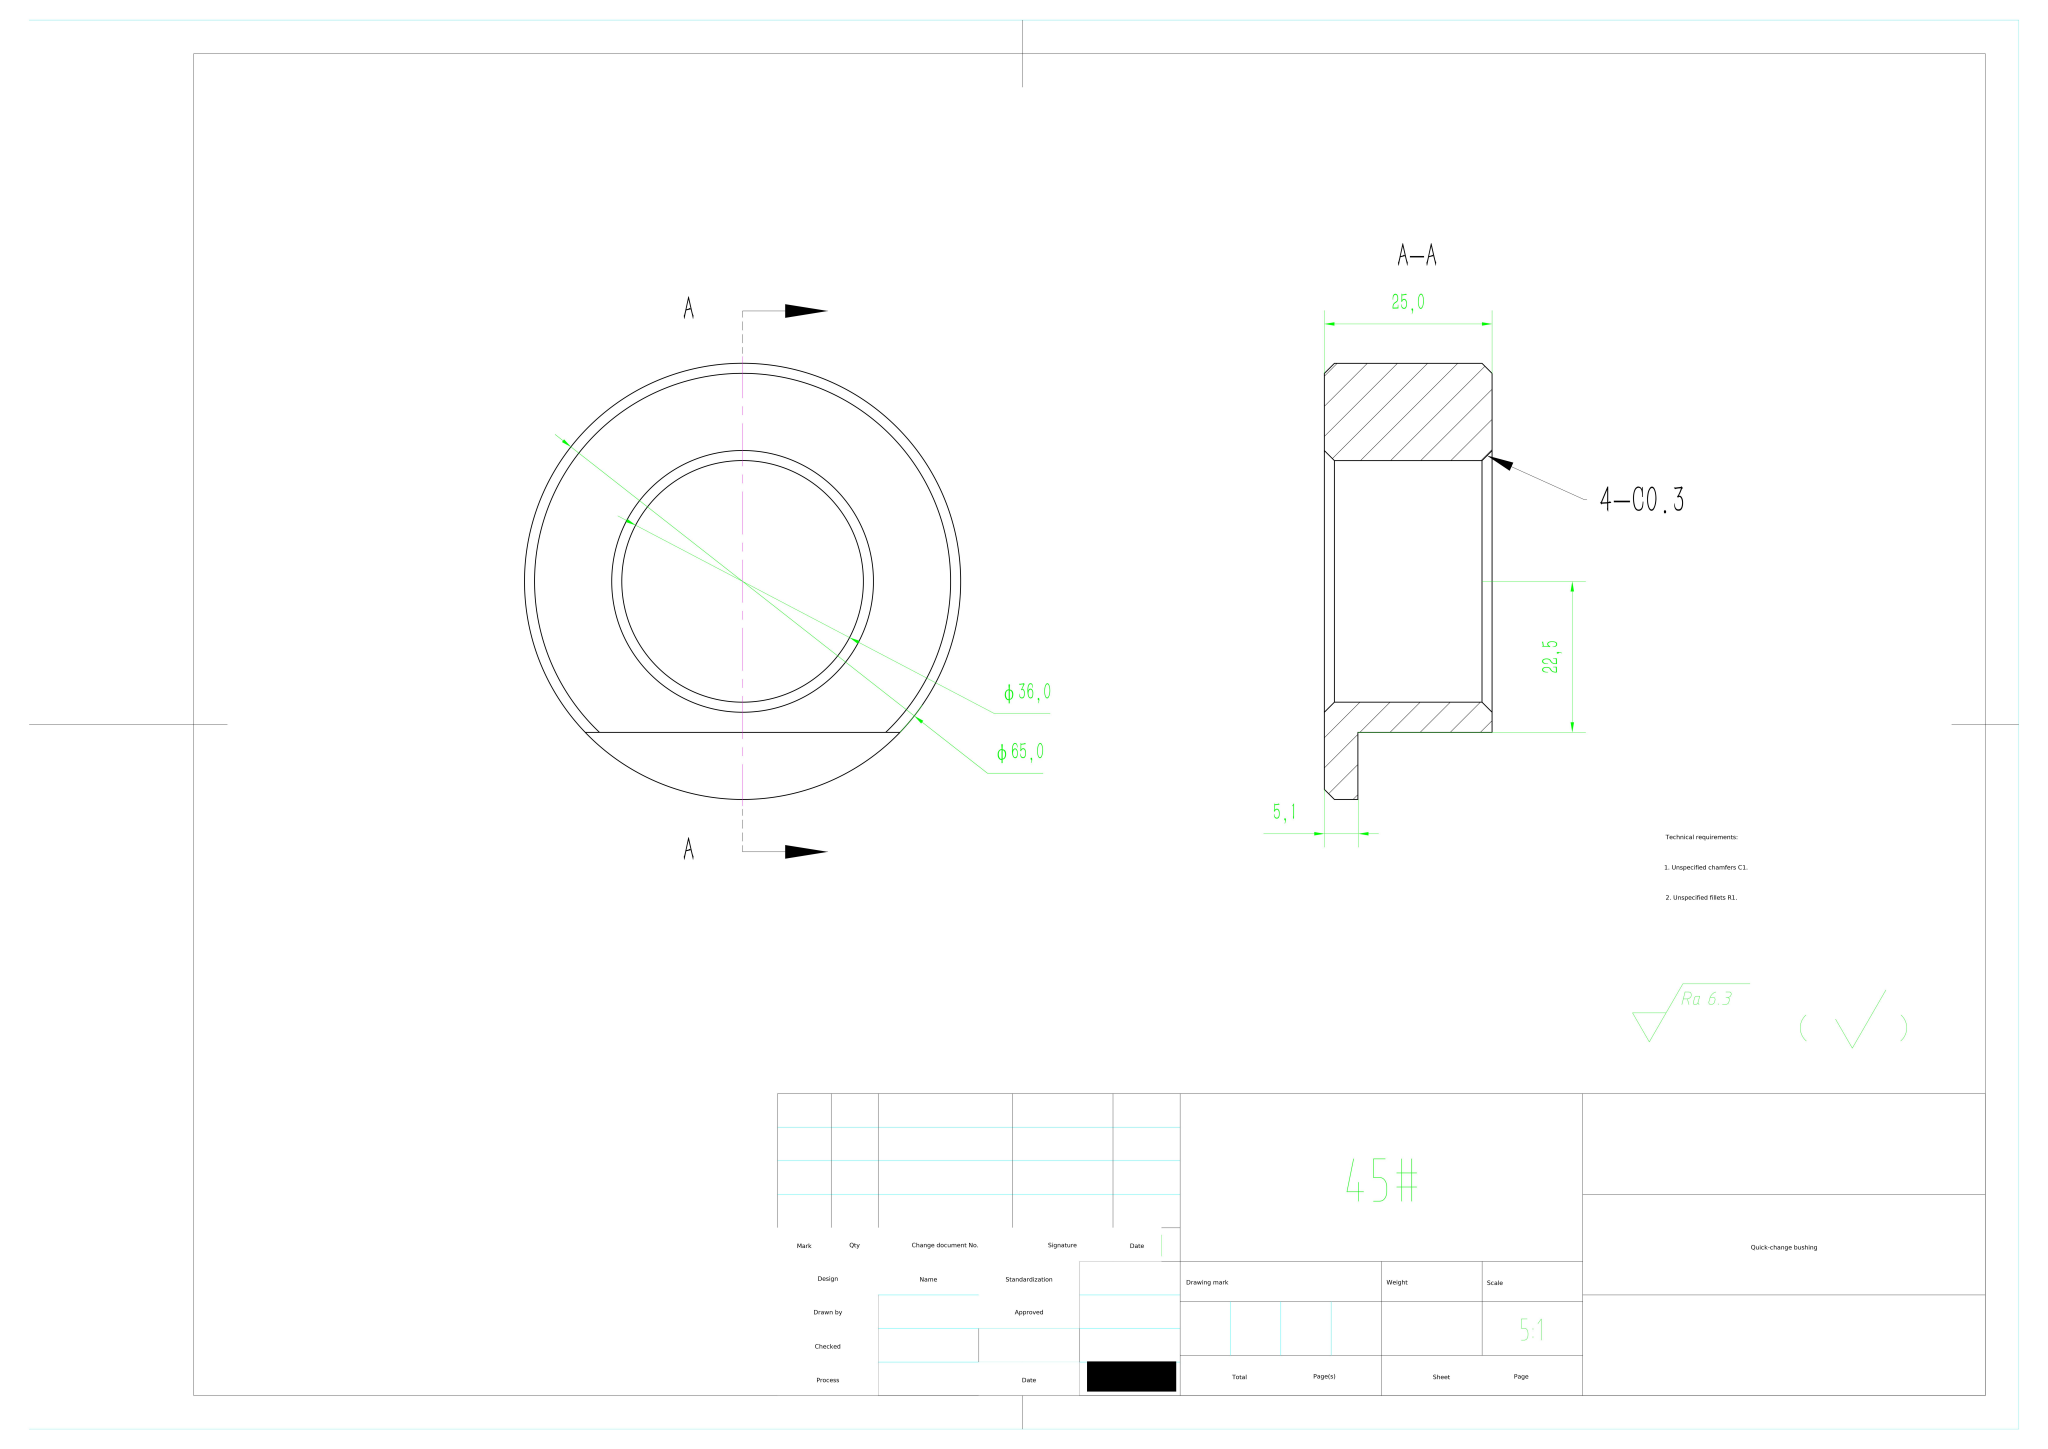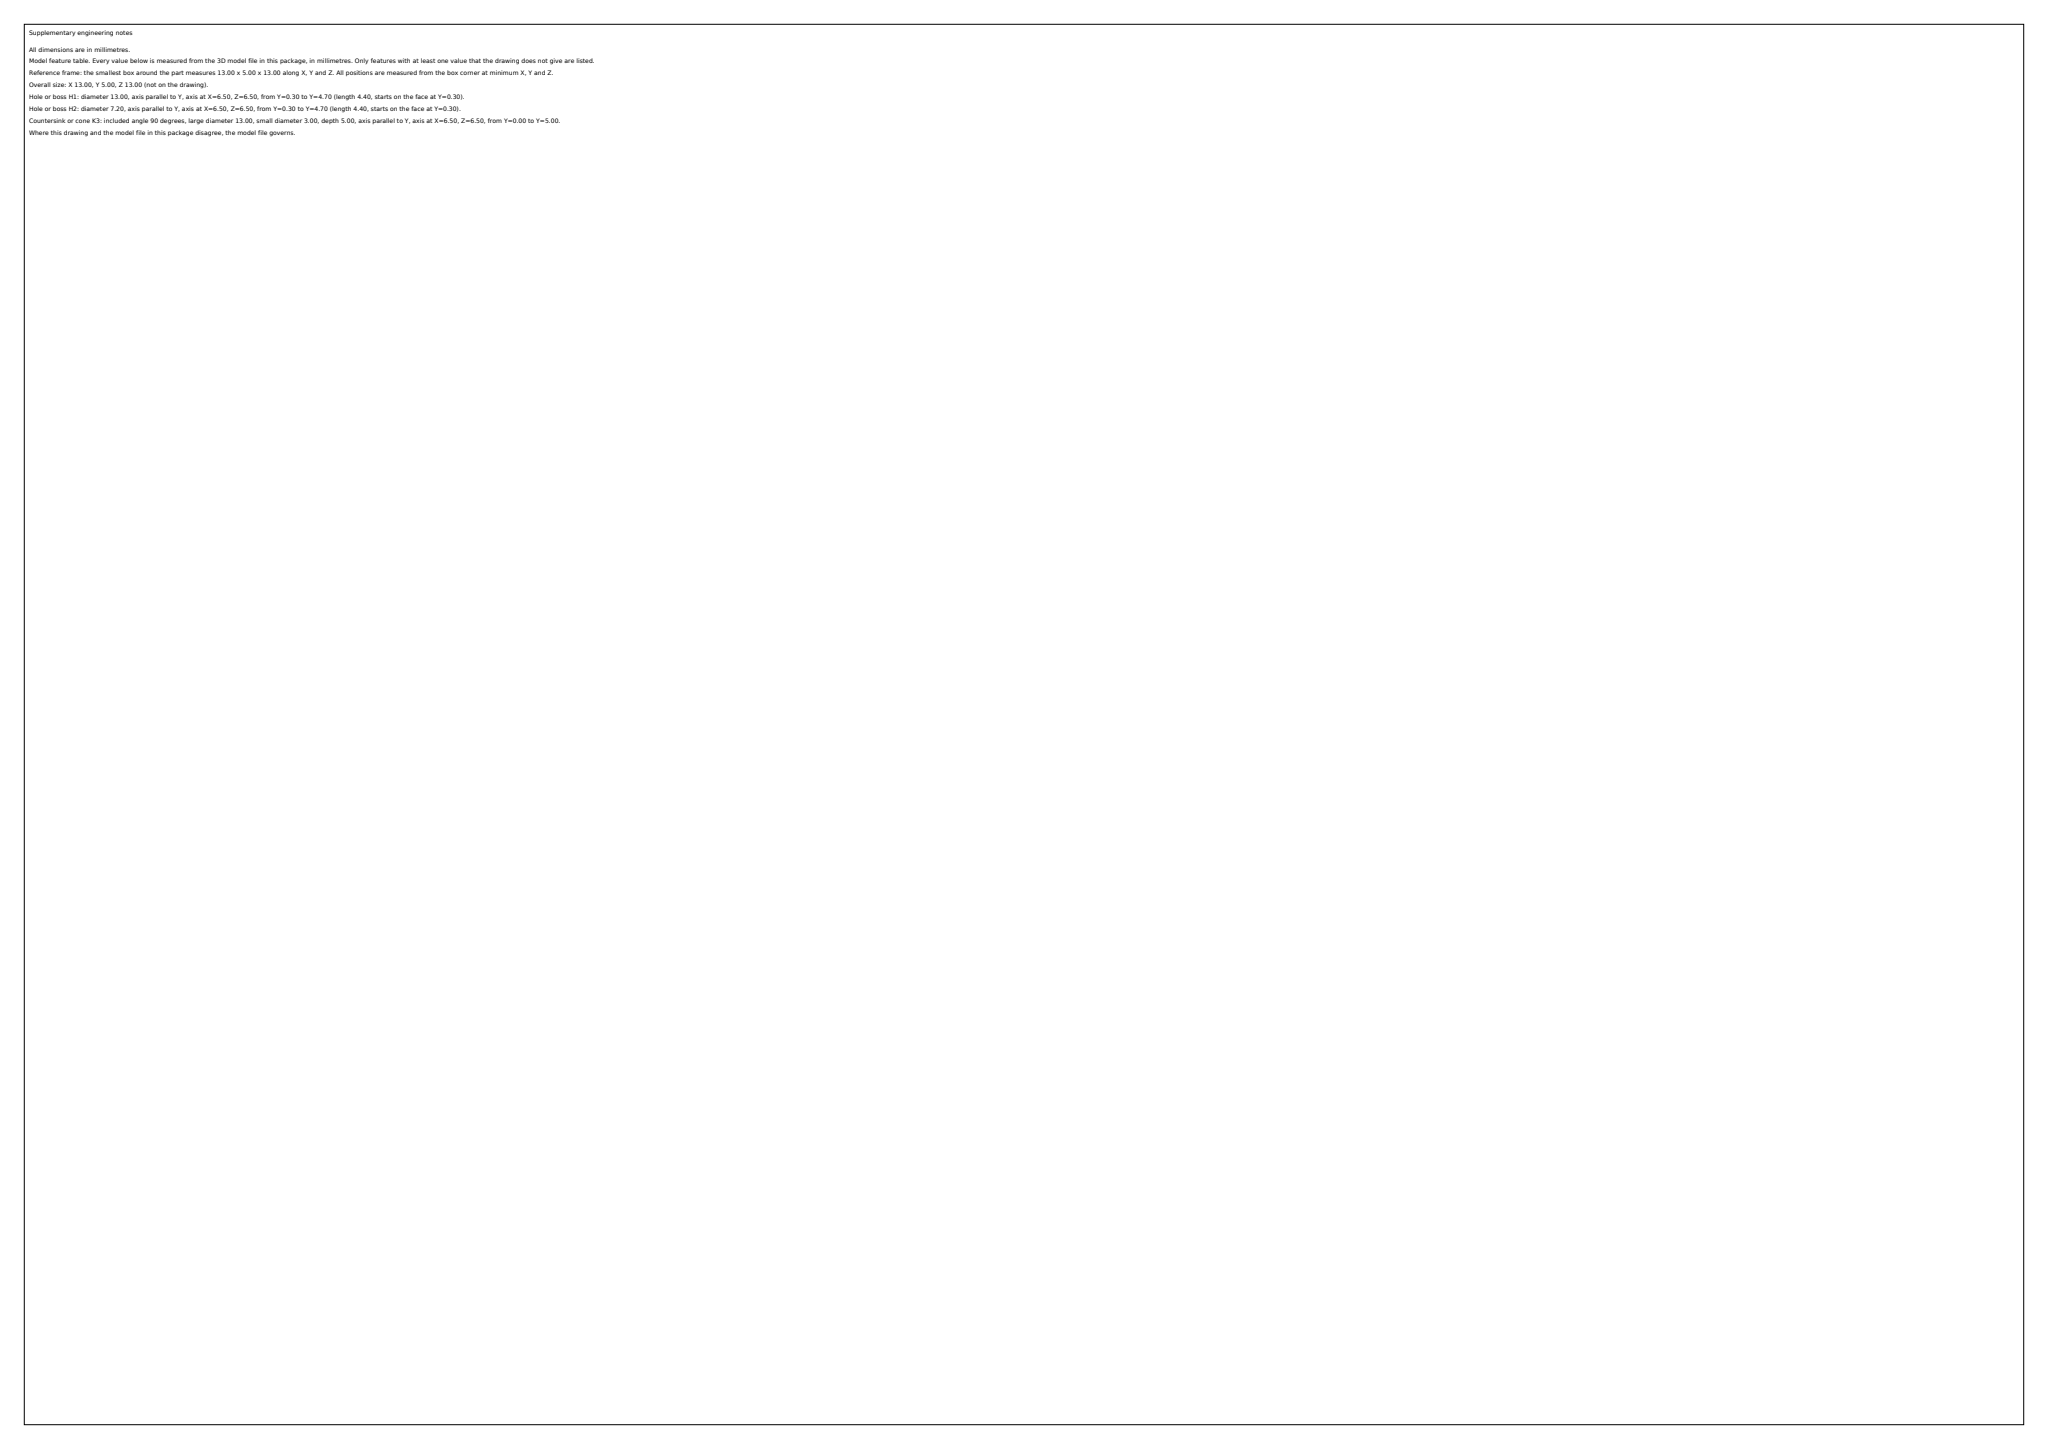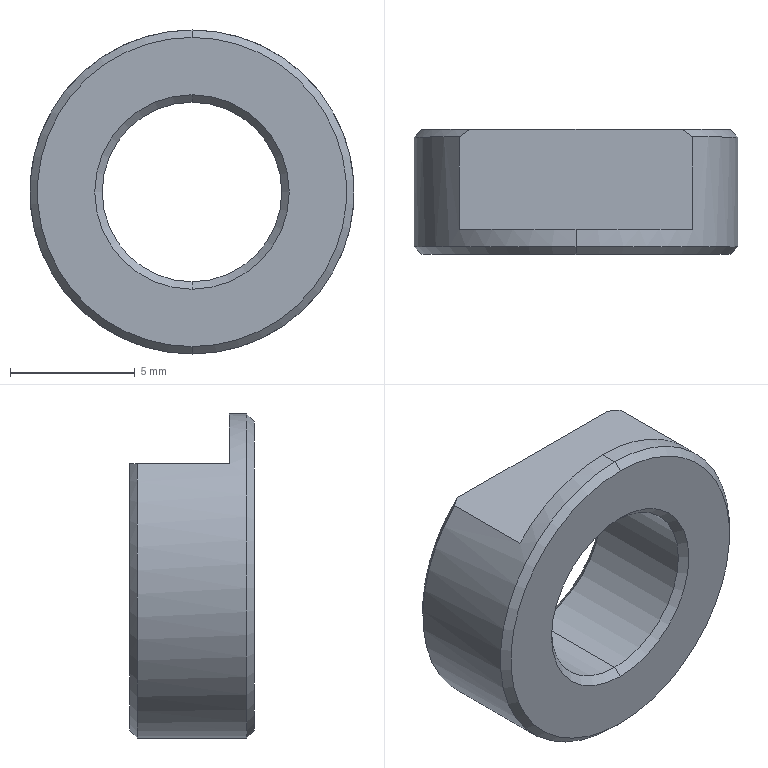Part | SolidWorks | mm | material 45# | 1 solid | 16 faces | box 13 x 5 x 13 mm | volume 403 mm3 | cone 8 | cylinder 4 | plane 4 | commonest cylinder face diameters 7.2 x2 13 x2
build123d program:
from build123d import *

# Parameters (mm, degrees)
SKETCH1_R           = 6.5
SKETCH1_R_2         = 3.6
BOSS_EXTRUDE1_DEPTH = 5
CHAMFER1_SIZE       = 0.3
SKETCH2_W           = 21.052
SKETCH2_H           = 6.896
CUT_EXTRUDE1_DEPTH  = 4


with BuildPart() as part:
    # Sketch1 → Boss-Extrude1 (new body)
    with BuildSketch(Plane(origin=(0, 0, 0), x_dir=(1, 0, 0), z_dir=(0, 1, 0))):
        with Locations(Location((0, 0, 0), (0, 0, 270))):
            Circle(SKETCH1_R)
        with Locations(Location((0, 0, 0), (0, 0, 270))):
            Circle(SKETCH1_R_2, mode=Mode.SUBTRACT)
    extrude(amount=BOSS_EXTRUDE1_DEPTH)

    # Chamfer1
    chamfer1_edges = [part.edges().sort_by_distance(p)[0] for p in [
        (0, 0, -6.5),
        (0, 5, -6.5),
        (0, 0, -3.6),
        (0, 5, -3.6),
    ]]
    chamfer(chamfer1_edges, length=CHAMFER1_SIZE)

    # Sketch2 → Cut-Extrude1 (cut)
    with BuildSketch(Plane(origin=(0, 5, 0), x_dir=(1, 0, 0), z_dir=(0, 1, 0))):
        with Locations((1.769, -7.948)):
            Rectangle(SKETCH2_W, SKETCH2_H)
    extrude(amount=-CUT_EXTRUDE1_DEPTH, mode=Mode.SUBTRACT)


solid = part.part
STEP:
#1=CARTESIAN_POINT('',(0.,5.,-6.2));
#2=VERTEX_POINT('',#1);
#3=CARTESIAN_POINT('',(-4.265,5.,4.5));
#4=VERTEX_POINT('',#3);
#5=CARTESIAN_POINT('',(0.,5.,0.));
#6=DIRECTION('',(0.,1.,0.));
#7=DIRECTION('',(0.,0.,1.));
#8=AXIS2_PLACEMENT_3D('',#5,#6,#7);
#9=CIRCLE('',#8,6.2);
#10=EDGE_CURVE('',#2,#4,#9,.T.);
#11=ORIENTED_EDGE('',*,*,#10,.F.);
#12=CARTESIAN_POINT('',(0.,4.7,-6.5));
#13=VERTEX_POINT('',#12);
#14=CARTESIAN_POINT('',(0.,5.,-6.2));
#15=DIRECTION('',(0.,-0.7071,-0.7071));
#16=VECTOR('',#15,1000.);
#17=LINE('',#14,#16);
#18=EDGE_CURVE('',#2,#13,#17,.T.);
#19=ORIENTED_EDGE('',*,*,#18,.T.);
#20=CARTESIAN_POINT('',(-4.69,4.7,4.5));
#21=VERTEX_POINT('',#20);
#22=CARTESIAN_POINT('',(0.,4.7,0.));
#23=DIRECTION('',(0.,-1.,0.));
#24=DIRECTION('',(0.,0.,1.));
#25=AXIS2_PLACEMENT_3D('',#22,#23,#24);
#26=CIRCLE('',#25,6.5);
#27=EDGE_CURVE('',#21,#13,#26,.T.);
#28=ORIENTED_EDGE('',*,*,#27,.F.);
#29=CARTESIAN_POINT('',(-4.265,5.,4.5));
#30=CARTESIAN_POINT('',(-4.408,4.902,4.5));
#31=CARTESIAN_POINT('',(-4.55,4.802,4.5));
#32=CARTESIAN_POINT('',(-4.69,4.7,4.5));
#33=B_SPLINE_CURVE_WITH_KNOTS('',3,(#29,#30,#31,#32),.UNSPECIFIED.,.F.,.F.,(4,4),(0.02154,0.02205),.UNSPECIFIED.);
#34=EDGE_CURVE('',#4,#21,#33,.T.);
#35=ORIENTED_EDGE('',*,*,#34,.F.);
#36=EDGE_LOOP('',(#11,#19,#28,#35));
#37=FACE_OUTER_BOUND('',#36,.T.);
#38=CARTESIAN_POINT('',(0.,5.,0.));
#39=DIRECTION('',(0.,-1.,0.));
#40=DIRECTION('',(0.,0.,-1.));
#41=AXIS2_PLACEMENT_3D('',#38,#39,#40);
#42=CONICAL_SURFACE('',#41,6.2,0.7854);
#43=ADVANCED_FACE('',(#37),#42,.T.);
#44=CARTESIAN_POINT('',(0.,4.7,-3.6));
#45=VERTEX_POINT('',#44);
#46=CARTESIAN_POINT('',(0.,4.7,3.6));
#47=VERTEX_POINT('',#46);
#48=CARTESIAN_POINT('',(0.,4.7,0.));
#49=DIRECTION('',(0.,1.,0.));
#50=DIRECTION('',(0.,0.,1.));
#51=AXIS2_PLACEMENT_3D('',#48,#49,#50);
#52=CIRCLE('',#51,3.6);
#53=EDGE_CURVE('',#45,#47,#52,.T.);
#54=ORIENTED_EDGE('',*,*,#53,.F.);
#55=CARTESIAN_POINT('',(0.,5.,-3.9));
#56=VERTEX_POINT('',#55);
#57=CARTESIAN_POINT('',(0.,4.7,-3.6));
#58=DIRECTION('',(0.,0.7071,-0.7071));
#59=VECTOR('',#58,1000.);
#60=LINE('',#57,#59);
#61=EDGE_CURVE('',#45,#56,#60,.T.);
#62=ORIENTED_EDGE('',*,*,#61,.T.);
#63=CARTESIAN_POINT('',(0.,5.,3.9));
#64=VERTEX_POINT('',#63);
#65=CARTESIAN_POINT('',(0.,5.,0.));
#66=DIRECTION('',(0.,-1.,0.));
#67=DIRECTION('',(0.,0.,1.));
#68=AXIS2_PLACEMENT_3D('',#65,#66,#67);
#69=CIRCLE('',#68,3.9);
#70=EDGE_CURVE('',#64,#56,#69,.T.);
#71=ORIENTED_EDGE('',*,*,#70,.F.);
#72=CARTESIAN_POINT('',(0.,4.7,3.6));
#73=DIRECTION('',(0.,0.7071,0.7071));
#74=VECTOR('',#73,1000.);
#75=LINE('',#72,#74);
#76=EDGE_CURVE('',#47,#64,#75,.T.);
#77=ORIENTED_EDGE('',*,*,#76,.F.);
#78=EDGE_LOOP('',(#54,#62,#71,#77));
#79=FACE_OUTER_BOUND('',#78,.T.);
#80=CARTESIAN_POINT('',(0.,4.7,0.));
#81=DIRECTION('',(0.,1.,0.));
#82=DIRECTION('',(0.,0.,1.));
#83=AXIS2_PLACEMENT_3D('',#80,#81,#82);
#84=CONICAL_SURFACE('',#83,3.6,0.7854);
#85=ADVANCED_FACE('',(#79),#84,.F.);
#86=CARTESIAN_POINT('',(0.,0.,-6.2));
#87=VERTEX_POINT('',#86);
#88=CARTESIAN_POINT('',(0.,0.,6.2));
#89=VERTEX_POINT('',#88);
#90=CARTESIAN_POINT('',(0.,0.,0.));
#91=DIRECTION('',(0.,-1.,0.));
#92=DIRECTION('',(0.,0.,1.));
#93=AXIS2_PLACEMENT_3D('',#90,#91,#92);
#94=CIRCLE('',#93,6.2);
#95=EDGE_CURVE('',#87,#89,#94,.T.);
#96=ORIENTED_EDGE('',*,*,#95,.F.);
#97=CARTESIAN_POINT('',(0.,0.3,-6.5));
#98=VERTEX_POINT('',#97);
#99=CARTESIAN_POINT('',(0.,0.3,-6.5));
#100=DIRECTION('',(0.,0.7071,-0.7071));
#101=VECTOR('',#100,1000.);
#102=LINE('',#99,#101);
#103=EDGE_CURVE('',#87,#98,#102,.T.);
#104=ORIENTED_EDGE('',*,*,#103,.T.);
#105=CARTESIAN_POINT('',(0.,0.3,6.5));
#106=VERTEX_POINT('',#105);
#107=CARTESIAN_POINT('',(0.,0.3,0.));
#108=DIRECTION('',(0.,1.,0.));
#109=DIRECTION('',(0.,0.,1.));
#110=AXIS2_PLACEMENT_3D('',#107,#108,#109);
#111=CIRCLE('',#110,6.5);
#112=EDGE_CURVE('',#106,#98,#111,.T.);
#113=ORIENTED_EDGE('',*,*,#112,.F.);
#114=CARTESIAN_POINT('',(0.,0.3,6.5));
#115=DIRECTION('',(0.,0.7071,0.7071));
#116=VECTOR('',#115,1000.);
#117=LINE('',#114,#116);
#118=EDGE_CURVE('',#89,#106,#117,.T.);
#119=ORIENTED_EDGE('',*,*,#118,.F.);
#120=EDGE_LOOP('',(#96,#104,#113,#119));
#121=FACE_OUTER_BOUND('',#120,.T.);
#122=CARTESIAN_POINT('',(0.,0.3,0.));
#123=DIRECTION('',(0.,1.,0.));
#124=DIRECTION('',(0.,0.,1.));
#125=AXIS2_PLACEMENT_3D('',#122,#123,#124);
#126=CONICAL_SURFACE('',#125,6.5,0.7854);
#127=ADVANCED_FACE('',(#121),#126,.T.);
#128=CARTESIAN_POINT('',(0.,0.3,3.6));
#129=VERTEX_POINT('',#128);
#130=CARTESIAN_POINT('',(0.,0.3,-3.6));
#131=VERTEX_POINT('',#130);
#132=CARTESIAN_POINT('',(0.,0.3,0.));
#133=DIRECTION('',(0.,-1.,0.));
#134=DIRECTION('',(0.,0.,1.));
#135=AXIS2_PLACEMENT_3D('',#132,#133,#134);
#136=CIRCLE('',#135,3.6);
#137=EDGE_CURVE('',#129,#131,#136,.T.);
#138=ORIENTED_EDGE('',*,*,#137,.F.);
#139=CARTESIAN_POINT('',(0.,0.,3.9));
#140=VERTEX_POINT('',#139);
#141=CARTESIAN_POINT('',(0.,0.,3.9));
#142=DIRECTION('',(0.,-0.7071,0.7071));
#143=VECTOR('',#142,1000.);
#144=LINE('',#141,#143);
#145=EDGE_CURVE('',#129,#140,#144,.T.);
#146=ORIENTED_EDGE('',*,*,#145,.T.);
#147=CARTESIAN_POINT('',(0.,0.,-3.9));
#148=VERTEX_POINT('',#147);
#149=CARTESIAN_POINT('',(0.,0.,0.));
#150=DIRECTION('',(0.,1.,0.));
#151=DIRECTION('',(0.,0.,1.));
#152=AXIS2_PLACEMENT_3D('',#149,#150,#151);
#153=CIRCLE('',#152,3.9);
#154=EDGE_CURVE('',#148,#140,#153,.T.);
#155=ORIENTED_EDGE('',*,*,#154,.F.);
#156=CARTESIAN_POINT('',(0.,0.,-3.9));
#157=DIRECTION('',(0.,-0.7071,-0.7071));
#158=VECTOR('',#157,1000.);
#159=LINE('',#156,#158);
#160=EDGE_CURVE('',#131,#148,#159,.T.);
#161=ORIENTED_EDGE('',*,*,#160,.F.);
#162=EDGE_LOOP('',(#138,#146,#155,#161));
#163=FACE_OUTER_BOUND('',#162,.T.);
#164=CARTESIAN_POINT('',(0.,0.,0.));
#165=DIRECTION('',(0.,-1.,0.));
#166=DIRECTION('',(0.,0.,-1.));
#167=AXIS2_PLACEMENT_3D('',#164,#165,#166);
#168=CONICAL_SURFACE('',#167,3.9,0.7854);
#169=ADVANCED_FACE('',(#163),#168,.F.);
#170=ORIENTED_EDGE('',*,*,#53,.T.);
#171=CARTESIAN_POINT('',(0.,5.,3.6));
#172=DIRECTION('',(0.,-1.,0.));
#173=VECTOR('',#172,1000.);
#174=LINE('',#171,#173);
#175=EDGE_CURVE('',#47,#129,#174,.T.);
#176=ORIENTED_EDGE('',*,*,#175,.T.);
#177=ORIENTED_EDGE('',*,*,#137,.T.);
#178=CARTESIAN_POINT('',(0.,5.,-3.6));
#179=DIRECTION('',(0.,-1.,0.));
#180=VECTOR('',#179,1000.);
#181=LINE('',#178,#180);
#182=EDGE_CURVE('',#45,#131,#181,.T.);
#183=ORIENTED_EDGE('',*,*,#182,.F.);
#184=EDGE_LOOP('',(#170,#176,#177,#183));
#185=FACE_OUTER_BOUND('',#184,.T.);
#186=CARTESIAN_POINT('',(0.,5.,0.));
#187=DIRECTION('',(0.,-1.,0.));
#188=DIRECTION('',(0.,0.,-1.));
#189=AXIS2_PLACEMENT_3D('',#186,#187,#188);
#190=CYLINDRICAL_SURFACE('',#189,3.6);
#191=ADVANCED_FACE('',(#185),#190,.F.);
#192=CARTESIAN_POINT('',(0.,1.,6.5));
#193=VERTEX_POINT('',#192);
#194=CARTESIAN_POINT('',(4.69,1.,4.5));
#195=VERTEX_POINT('',#194);
#196=CARTESIAN_POINT('',(0.,1.,0.));
#197=DIRECTION('',(0.,1.,0.));
#198=DIRECTION('',(0.,0.,1.));
#199=AXIS2_PLACEMENT_3D('',#196,#197,#198);
#200=CIRCLE('',#199,6.5);
#201=EDGE_CURVE('',#193,#195,#200,.T.);
#202=ORIENTED_EDGE('',*,*,#201,.F.);
#203=CARTESIAN_POINT('',(0.,5.,6.5));
#204=DIRECTION('',(0.,-1.,0.));
#205=VECTOR('',#204,1000.);
#206=LINE('',#203,#205);
#207=EDGE_CURVE('',#193,#106,#206,.T.);
#208=ORIENTED_EDGE('',*,*,#207,.T.);
#209=ORIENTED_EDGE('',*,*,#112,.T.);
#210=CARTESIAN_POINT('',(0.,5.,-6.5));
#211=DIRECTION('',(0.,-1.,0.));
#212=VECTOR('',#211,1000.);
#213=LINE('',#210,#212);
#214=EDGE_CURVE('',#13,#98,#213,.T.);
#215=ORIENTED_EDGE('',*,*,#214,.F.);
#216=CARTESIAN_POINT('',(4.69,4.7,4.5));
#217=VERTEX_POINT('',#216);
#218=CARTESIAN_POINT('',(0.,4.7,0.));
#219=DIRECTION('',(0.,-1.,0.));
#220=DIRECTION('',(0.,0.,1.));
#221=AXIS2_PLACEMENT_3D('',#218,#219,#220);
#222=CIRCLE('',#221,6.5);
#223=EDGE_CURVE('',#13,#217,#222,.T.);
#224=ORIENTED_EDGE('',*,*,#223,.T.);
#225=CARTESIAN_POINT('',(4.69,5.,4.5));
#226=DIRECTION('',(0.,-1.,0.));
#227=VECTOR('',#226,1000.);
#228=LINE('',#225,#227);
#229=EDGE_CURVE('',#217,#195,#228,.T.);
#230=ORIENTED_EDGE('',*,*,#229,.T.);
#231=EDGE_LOOP('',(#202,#208,#209,#215,#224,#230));
#232=FACE_OUTER_BOUND('',#231,.T.);
#233=CARTESIAN_POINT('',(0.,5.,0.));
#234=DIRECTION('',(0.,-1.,0.));
#235=DIRECTION('',(0.,0.,-1.));
#236=AXIS2_PLACEMENT_3D('',#233,#234,#235);
#237=CYLINDRICAL_SURFACE('',#236,6.5);
#238=ADVANCED_FACE('',(#232),#237,.T.);
#239=CARTESIAN_POINT('',(4.265,5.,4.5));
#240=VERTEX_POINT('',#239);
#241=CARTESIAN_POINT('',(-8.756,5.,4.5));
#242=DIRECTION('',(-1.,0.,0.));
#243=VECTOR('',#242,1000.);
#244=LINE('',#241,#243);
#245=EDGE_CURVE('',#240,#4,#244,.T.);
#246=ORIENTED_EDGE('',*,*,#245,.F.);
#247=CARTESIAN_POINT('',(0.,5.,0.));
#248=DIRECTION('',(0.,1.,0.));
#249=DIRECTION('',(0.,0.,1.));
#250=AXIS2_PLACEMENT_3D('',#247,#248,#249);
#251=CIRCLE('',#250,6.2);
#252=EDGE_CURVE('',#240,#2,#251,.T.);
#253=ORIENTED_EDGE('',*,*,#252,.T.);
#254=ORIENTED_EDGE('',*,*,#10,.T.);
#255=EDGE_LOOP('',(#246,#253,#254));
#256=FACE_OUTER_BOUND('',#255,.T.);
#257=ORIENTED_EDGE('',*,*,#70,.T.);
#258=CARTESIAN_POINT('',(0.,5.,0.));
#259=DIRECTION('',(0.,-1.,0.));
#260=DIRECTION('',(0.,0.,1.));
#261=AXIS2_PLACEMENT_3D('',#258,#259,#260);
#262=CIRCLE('',#261,3.9);
#263=EDGE_CURVE('',#56,#64,#262,.T.);
#264=ORIENTED_EDGE('',*,*,#263,.T.);
#265=EDGE_LOOP('',(#257,#264));
#266=FACE_BOUND('',#265,.T.);
#267=CARTESIAN_POINT('',(0.,5.,0.));
#268=DIRECTION('',(0.,1.,0.));
#269=DIRECTION('',(0.,0.,1.));
#270=AXIS2_PLACEMENT_3D('',#267,#268,#269);
#271=PLANE('',#270);
#272=ADVANCED_FACE('',(#256,#266),#271,.T.);
#273=ORIENTED_EDGE('',*,*,#154,.T.);
#274=CARTESIAN_POINT('',(0.,0.,0.));
#275=DIRECTION('',(0.,1.,0.));
#276=DIRECTION('',(0.,0.,1.));
#277=AXIS2_PLACEMENT_3D('',#274,#275,#276);
#278=CIRCLE('',#277,3.9);
#279=EDGE_CURVE('',#140,#148,#278,.T.);
#280=ORIENTED_EDGE('',*,*,#279,.T.);
#281=EDGE_LOOP('',(#273,#280));
#282=FACE_BOUND('',#281,.T.);
#283=CARTESIAN_POINT('',(0.,0.,0.));
#284=DIRECTION('',(0.,-1.,0.));
#285=DIRECTION('',(0.,0.,1.));
#286=AXIS2_PLACEMENT_3D('',#283,#284,#285);
#287=CIRCLE('',#286,6.2);
#288=EDGE_CURVE('',#89,#87,#287,.T.);
#289=ORIENTED_EDGE('',*,*,#288,.T.);
#290=ORIENTED_EDGE('',*,*,#95,.T.);
#291=EDGE_LOOP('',(#289,#290));
#292=FACE_OUTER_BOUND('',#291,.T.);
#293=CARTESIAN_POINT('',(0.,0.,0.));
#294=DIRECTION('',(0.,1.,0.));
#295=DIRECTION('',(0.,0.,1.));
#296=AXIS2_PLACEMENT_3D('',#293,#294,#295);
#297=PLANE('',#296);
#298=ADVANCED_FACE('',(#282,#292),#297,.F.);
#299=ORIENTED_EDGE('',*,*,#207,.F.);
#300=CARTESIAN_POINT('',(-4.69,1.,4.5));
#301=VERTEX_POINT('',#300);
#302=CARTESIAN_POINT('',(0.,1.,0.));
#303=DIRECTION('',(0.,1.,0.));
#304=DIRECTION('',(0.,0.,1.));
#305=AXIS2_PLACEMENT_3D('',#302,#303,#304);
#306=CIRCLE('',#305,6.5);
#307=EDGE_CURVE('',#301,#193,#306,.T.);
#308=ORIENTED_EDGE('',*,*,#307,.F.);
#309=CARTESIAN_POINT('',(-4.69,5.,4.5));
#310=DIRECTION('',(0.,1.,0.));
#311=VECTOR('',#310,1000.);
#312=LINE('',#309,#311);
#313=EDGE_CURVE('',#301,#21,#312,.T.);
#314=ORIENTED_EDGE('',*,*,#313,.T.);
#315=ORIENTED_EDGE('',*,*,#27,.T.);
#316=ORIENTED_EDGE('',*,*,#214,.T.);
#317=CARTESIAN_POINT('',(0.,0.3,0.));
#318=DIRECTION('',(0.,1.,0.));
#319=DIRECTION('',(0.,0.,1.));
#320=AXIS2_PLACEMENT_3D('',#317,#318,#319);
#321=CIRCLE('',#320,6.5);
#322=EDGE_CURVE('',#98,#106,#321,.T.);
#323=ORIENTED_EDGE('',*,*,#322,.T.);
#324=EDGE_LOOP('',(#299,#308,#314,#315,#316,#323));
#325=FACE_OUTER_BOUND('',#324,.T.);
#326=CARTESIAN_POINT('',(0.,5.,0.));
#327=DIRECTION('',(0.,-1.,0.));
#328=DIRECTION('',(0.,0.,-1.));
#329=AXIS2_PLACEMENT_3D('',#326,#327,#328);
#330=CYLINDRICAL_SURFACE('',#329,6.5);
#331=ADVANCED_FACE('',(#325),#330,.T.);
#332=ORIENTED_EDGE('',*,*,#175,.F.);
#333=CARTESIAN_POINT('',(0.,4.7,0.));
#334=DIRECTION('',(0.,1.,0.));
#335=DIRECTION('',(0.,0.,1.));
#336=AXIS2_PLACEMENT_3D('',#333,#334,#335);
#337=CIRCLE('',#336,3.6);
#338=EDGE_CURVE('',#47,#45,#337,.T.);
#339=ORIENTED_EDGE('',*,*,#338,.T.);
#340=ORIENTED_EDGE('',*,*,#182,.T.);
#341=CARTESIAN_POINT('',(0.,0.3,0.));
#342=DIRECTION('',(0.,-1.,0.));
#343=DIRECTION('',(0.,0.,1.));
#344=AXIS2_PLACEMENT_3D('',#341,#342,#343);
#345=CIRCLE('',#344,3.6);
#346=EDGE_CURVE('',#131,#129,#345,.T.);
#347=ORIENTED_EDGE('',*,*,#346,.T.);
#348=EDGE_LOOP('',(#332,#339,#340,#347));
#349=FACE_OUTER_BOUND('',#348,.T.);
#350=CARTESIAN_POINT('',(0.,5.,0.));
#351=DIRECTION('',(0.,-1.,0.));
#352=DIRECTION('',(0.,0.,-1.));
#353=AXIS2_PLACEMENT_3D('',#350,#351,#352);
#354=CYLINDRICAL_SURFACE('',#353,3.6);
#355=ADVANCED_FACE('',(#349),#354,.F.);
#356=ORIENTED_EDGE('',*,*,#145,.F.);
#357=ORIENTED_EDGE('',*,*,#346,.F.);
#358=ORIENTED_EDGE('',*,*,#160,.T.);
#359=ORIENTED_EDGE('',*,*,#279,.F.);
#360=EDGE_LOOP('',(#356,#357,#358,#359));
#361=FACE_OUTER_BOUND('',#360,.T.);
#362=CARTESIAN_POINT('',(0.,0.,0.));
#363=DIRECTION('',(0.,-1.,0.));
#364=DIRECTION('',(0.,0.,-1.));
#365=AXIS2_PLACEMENT_3D('',#362,#363,#364);
#366=CONICAL_SURFACE('',#365,3.9,0.7854);
#367=ADVANCED_FACE('',(#361),#366,.F.);
#368=ORIENTED_EDGE('',*,*,#103,.F.);
#369=ORIENTED_EDGE('',*,*,#288,.F.);
#370=ORIENTED_EDGE('',*,*,#118,.T.);
#371=ORIENTED_EDGE('',*,*,#322,.F.);
#372=EDGE_LOOP('',(#368,#369,#370,#371));
#373=FACE_OUTER_BOUND('',#372,.T.);
#374=CARTESIAN_POINT('',(0.,0.3,0.));
#375=DIRECTION('',(0.,1.,0.));
#376=DIRECTION('',(0.,0.,1.));
#377=AXIS2_PLACEMENT_3D('',#374,#375,#376);
#378=CONICAL_SURFACE('',#377,6.5,0.7854);
#379=ADVANCED_FACE('',(#373),#378,.T.);
#380=ORIENTED_EDGE('',*,*,#61,.F.);
#381=ORIENTED_EDGE('',*,*,#338,.F.);
#382=ORIENTED_EDGE('',*,*,#76,.T.);
#383=ORIENTED_EDGE('',*,*,#263,.F.);
#384=EDGE_LOOP('',(#380,#381,#382,#383));
#385=FACE_OUTER_BOUND('',#384,.T.);
#386=CARTESIAN_POINT('',(0.,4.7,0.));
#387=DIRECTION('',(0.,1.,0.));
#388=DIRECTION('',(0.,0.,1.));
#389=AXIS2_PLACEMENT_3D('',#386,#387,#388);
#390=CONICAL_SURFACE('',#389,3.6,0.7854);
#391=ADVANCED_FACE('',(#385),#390,.F.);
#392=ORIENTED_EDGE('',*,*,#18,.F.);
#393=ORIENTED_EDGE('',*,*,#252,.F.);
#394=CARTESIAN_POINT('',(4.69,4.7,4.5));
#395=CARTESIAN_POINT('',(4.55,4.802,4.5));
#396=CARTESIAN_POINT('',(4.408,4.902,4.5));
#397=CARTESIAN_POINT('',(4.265,5.,4.5));
#398=B_SPLINE_CURVE_WITH_KNOTS('',3,(#394,#395,#396,#397),.UNSPECIFIED.,.F.,.F.,(4,4),(0.01184,0.01237),.UNSPECIFIED.);
#399=EDGE_CURVE('',#217,#240,#398,.T.);
#400=ORIENTED_EDGE('',*,*,#399,.F.);
#401=ORIENTED_EDGE('',*,*,#223,.F.);
#402=EDGE_LOOP('',(#392,#393,#400,#401));
#403=FACE_OUTER_BOUND('',#402,.T.);
#404=CARTESIAN_POINT('',(0.,5.,0.));
#405=DIRECTION('',(0.,-1.,0.));
#406=DIRECTION('',(0.,0.,-1.));
#407=AXIS2_PLACEMENT_3D('',#404,#405,#406);
#408=CONICAL_SURFACE('',#407,6.2,0.7854);
#409=ADVANCED_FACE('',(#403),#408,.T.);
#410=ORIENTED_EDGE('',*,*,#307,.T.);
#411=ORIENTED_EDGE('',*,*,#201,.T.);
#412=CARTESIAN_POINT('',(-8.756,1.,4.5));
#413=DIRECTION('',(-1.,0.,0.));
#414=VECTOR('',#413,1000.);
#415=LINE('',#412,#414);
#416=EDGE_CURVE('',#195,#301,#415,.T.);
#417=ORIENTED_EDGE('',*,*,#416,.T.);
#418=EDGE_LOOP('',(#410,#411,#417));
#419=FACE_OUTER_BOUND('',#418,.T.);
#420=CARTESIAN_POINT('',(0.,1.,0.));
#421=DIRECTION('',(0.,1.,0.));
#422=DIRECTION('',(0.,0.,1.));
#423=AXIS2_PLACEMENT_3D('',#420,#421,#422);
#424=PLANE('',#423);
#425=ADVANCED_FACE('',(#419),#424,.T.);
#426=ORIENTED_EDGE('',*,*,#399,.T.);
#427=ORIENTED_EDGE('',*,*,#245,.T.);
#428=ORIENTED_EDGE('',*,*,#34,.T.);
#429=ORIENTED_EDGE('',*,*,#313,.F.);
#430=ORIENTED_EDGE('',*,*,#416,.F.);
#431=ORIENTED_EDGE('',*,*,#229,.F.);
#432=EDGE_LOOP('',(#426,#427,#428,#429,#430,#431));
#433=FACE_OUTER_BOUND('',#432,.T.);
#434=CARTESIAN_POINT('',(-8.756,1.,4.5));
#435=DIRECTION('',(0.,0.,-1.));
#436=DIRECTION('',(-1.,0.,0.));
#437=AXIS2_PLACEMENT_3D('',#434,#435,#436);
#438=PLANE('',#437);
#439=ADVANCED_FACE('',(#433),#438,.F.);
#440=CLOSED_SHELL('',(#43,#85,#127,#169,#191,#238,#272,#298,#331,#355,#367,#379,#391,#409,#425,#439));
#441=MANIFOLD_SOLID_BREP('',#440);
#442=CARTESIAN_POINT('',(0.,0.,0.));
#443=DIRECTION('',(0.,0.,1.));
#444=DIRECTION('',(1.,0.,0.));
#445=AXIS2_PLACEMENT_3D('',#442,#443,#444);
#446=(LENGTH_UNIT()NAMED_UNIT(*)SI_UNIT(.MILLI.,.METRE.));
#447=UNCERTAINTY_MEASURE_WITH_UNIT(LENGTH_MEASURE(0.00001),#446,'','');
#448=(NAMED_UNIT(*)PLANE_ANGLE_UNIT()SI_UNIT($,.RADIAN.));
#449=(NAMED_UNIT(*)SI_UNIT($,.STERADIAN.)SOLID_ANGLE_UNIT());
#450=(GEOMETRIC_REPRESENTATION_CONTEXT(3)GLOBAL_UNCERTAINTY_ASSIGNED_CONTEXT((#447))GLOBAL_UNIT_ASSIGNED_CONTEXT((#446,#448,#449))REPRESENTATION_CONTEXT('',''));
#451=ADVANCED_BREP_SHAPE_REPRESENTATION('',(#441,#445),#450);